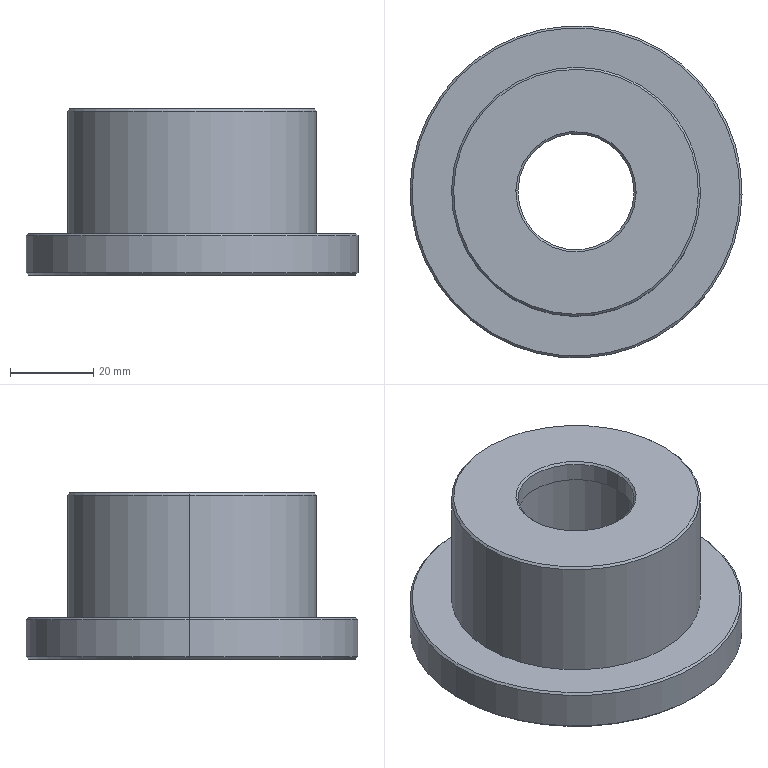Component | SolidWorks | HopperAssembly-1_20211103-210426-70669.STEP-1_-_-_-1.STEP-1_-_-_-4.STEP-1 | 1 solid | 34 faces | box 80 x 80 x 40 mm | volume 97628 mm3 | cylinder 16 | cone 10 | plane 8 | commonest cylinder face diameters 35 x6 39.6 x2 60 x2 80 x2 37 x2 28 x2
STEP:
#1=COLOUR_RGB('',0.7922,0.8196,0.9333);
#2=FILL_AREA_STYLE_COLOUR('',#1);
#3=FILL_AREA_STYLE('',(#2));
#4=SURFACE_STYLE_FILL_AREA(#3);
#5=SURFACE_SIDE_STYLE('',(#4));
#6=SURFACE_STYLE_USAGE(.BOTH.,#5);
#7=PRESENTATION_STYLE_ASSIGNMENT((#6));
#8=CARTESIAN_POINT('',(-116.904,33.244,9.945));
#9=VERTEX_POINT('',#8);
#10=CARTESIAN_POINT('',(-115.526,33.22,9.945));
#11=VERTEX_POINT('',#10);
#12=CARTESIAN_POINT('',(-116.215,33.232,9.945));
#13=DIRECTION('',(0.,0.,-1.));
#14=DIRECTION('',(-0.9998,0.01747,0.));
#15=AXIS2_PLACEMENT_3D('',#12,#13,#14);
#16=CIRCLE('',#15,0.689);
#17=EDGE_CURVE('',#9,#11,#16,.T.);
#18=ORIENTED_EDGE('',*,*,#17,.T.);
#19=CARTESIAN_POINT('',(-115.526,33.22,10.733));
#20=VERTEX_POINT('',#19);
#21=CARTESIAN_POINT('',(-115.526,33.22,10.93));
#22=DIRECTION('',(-0.,-0.,1.));
#23=VECTOR('',#22,39.37);
#24=LINE('',#21,#23);
#25=EDGE_CURVE('',#11,#20,#24,.T.);
#26=ORIENTED_EDGE('',*,*,#25,.T.);
#27=CARTESIAN_POINT('',(-116.904,33.244,10.733));
#28=VERTEX_POINT('',#27);
#29=CARTESIAN_POINT('',(-116.215,33.232,10.733));
#30=DIRECTION('',(-0.,-0.,1.));
#31=DIRECTION('',(-0.9998,0.01747,0.));
#32=AXIS2_PLACEMENT_3D('',#29,#30,#31);
#33=CIRCLE('',#32,0.689);
#34=EDGE_CURVE('',#20,#28,#33,.T.);
#35=ORIENTED_EDGE('',*,*,#34,.T.);
#36=CARTESIAN_POINT('',(-116.904,33.244,10.93));
#37=DIRECTION('',(-0.,-0.,1.));
#38=VECTOR('',#37,39.37);
#39=LINE('',#36,#38);
#40=EDGE_CURVE('',#9,#28,#39,.T.);
#41=ORIENTED_EDGE('',*,*,#40,.F.);
#42=EDGE_LOOP('',(#18,#26,#35,#41));
#43=FACE_OUTER_BOUND('',#42,.T.);
#44=CARTESIAN_POINT('',(-116.215,33.232,10.93));
#45=DIRECTION('',(-0.,-0.,1.));
#46=DIRECTION('',(-0.9998,0.01747,0.));
#47=AXIS2_PLACEMENT_3D('',#44,#45,#46);
#48=CYLINDRICAL_SURFACE('',#47,0.689);
#49=ADVANCED_FACE('',(#43),#48,.F.);
#50=CARTESIAN_POINT('',(-115.436,33.218,9.886));
#51=VERTEX_POINT('',#50);
#52=CARTESIAN_POINT('',(-116.995,33.245,9.886));
#53=VERTEX_POINT('',#52);
#54=CARTESIAN_POINT('',(-116.215,33.232,9.886));
#55=DIRECTION('',(-0.,-0.,1.));
#56=DIRECTION('',(-0.9998,0.01747,0.));
#57=AXIS2_PLACEMENT_3D('',#54,#55,#56);
#58=CIRCLE('',#57,0.7795);
#59=EDGE_CURVE('',#51,#53,#58,.T.);
#60=ORIENTED_EDGE('',*,*,#59,.F.);
#61=CARTESIAN_POINT('',(-115.436,33.218,9.945));
#62=VERTEX_POINT('',#61);
#63=CARTESIAN_POINT('',(-115.436,33.218,11.52));
#64=DIRECTION('',(-0.,-0.,1.));
#65=VECTOR('',#64,39.37);
#66=LINE('',#63,#65);
#67=EDGE_CURVE('',#51,#62,#66,.T.);
#68=ORIENTED_EDGE('',*,*,#67,.T.);
#69=CARTESIAN_POINT('',(-116.995,33.245,9.945));
#70=VERTEX_POINT('',#69);
#71=CARTESIAN_POINT('',(-116.215,33.232,9.945));
#72=DIRECTION('',(-0.,-0.,1.));
#73=DIRECTION('',(-0.9998,0.01747,0.));
#74=AXIS2_PLACEMENT_3D('',#71,#72,#73);
#75=CIRCLE('',#74,0.7795);
#76=EDGE_CURVE('',#62,#70,#75,.T.);
#77=ORIENTED_EDGE('',*,*,#76,.T.);
#78=CARTESIAN_POINT('',(-116.995,33.245,11.52));
#79=DIRECTION('',(-0.,-0.,1.));
#80=VECTOR('',#79,39.37);
#81=LINE('',#78,#80);
#82=EDGE_CURVE('',#53,#70,#81,.T.);
#83=ORIENTED_EDGE('',*,*,#82,.F.);
#84=EDGE_LOOP('',(#60,#68,#77,#83));
#85=FACE_OUTER_BOUND('',#84,.T.);
#86=CARTESIAN_POINT('',(-116.215,33.232,11.52));
#87=DIRECTION('',(-0.,-0.,1.));
#88=DIRECTION('',(-0.9998,0.01747,0.));
#89=AXIS2_PLACEMENT_3D('',#86,#87,#88);
#90=CYLINDRICAL_SURFACE('',#89,0.7795);
#91=ADVANCED_FACE('',(#85),#90,.F.);
#92=CARTESIAN_POINT('',(-117.77,33.259,9.749));
#93=VERTEX_POINT('',#92);
#94=CARTESIAN_POINT('',(-117.79,33.259,9.729));
#95=VERTEX_POINT('',#94);
#96=CARTESIAN_POINT('',(-117.77,33.259,9.749));
#97=DIRECTION('',(-0.707,0.01235,-0.7071));
#98=VECTOR('',#97,39.37);
#99=LINE('',#96,#98);
#100=EDGE_CURVE('',#93,#95,#99,.T.);
#101=ORIENTED_EDGE('',*,*,#100,.F.);
#102=CARTESIAN_POINT('',(-114.66,33.205,9.749));
#103=VERTEX_POINT('',#102);
#104=CARTESIAN_POINT('',(-116.215,33.232,9.749));
#105=DIRECTION('',(-0.,-0.,1.));
#106=DIRECTION('',(0.9998,-0.01747,0.));
#107=AXIS2_PLACEMENT_3D('',#104,#105,#106);
#108=CIRCLE('',#107,1.555);
#109=EDGE_CURVE('',#103,#93,#108,.T.);
#110=ORIENTED_EDGE('',*,*,#109,.F.);
#111=CARTESIAN_POINT('',(-114.641,33.204,9.729));
#112=VERTEX_POINT('',#111);
#113=CARTESIAN_POINT('',(-114.66,33.205,9.749));
#114=DIRECTION('',(0.707,-0.01235,-0.7071));
#115=VECTOR('',#114,39.37);
#116=LINE('',#113,#115);
#117=EDGE_CURVE('',#103,#112,#116,.T.);
#118=ORIENTED_EDGE('',*,*,#117,.T.);
#119=CARTESIAN_POINT('',(-116.215,33.232,9.729));
#120=DIRECTION('',(0.,0.,-1.));
#121=DIRECTION('',(0.9998,-0.01747,0.));
#122=AXIS2_PLACEMENT_3D('',#119,#120,#121);
#123=CIRCLE('',#122,1.575);
#124=EDGE_CURVE('',#95,#112,#123,.T.);
#125=ORIENTED_EDGE('',*,*,#124,.F.);
#126=EDGE_LOOP('',(#101,#110,#118,#125));
#127=FACE_OUTER_BOUND('',#126,.T.);
#128=CARTESIAN_POINT('',(-116.215,33.232,9.749));
#129=DIRECTION('',(0.,0.,-1.));
#130=DIRECTION('',(0.9998,-0.01747,0.));
#131=AXIS2_PLACEMENT_3D('',#128,#129,#130);
#132=CONICAL_SURFACE('',#131,1.555,0.7854);
#133=ADVANCED_FACE('',(#127),#132,.T.);
#134=CARTESIAN_POINT('',(-114.66,33.205,9.355));
#135=VERTEX_POINT('',#134);
#136=CARTESIAN_POINT('',(-114.641,33.204,9.375));
#137=VERTEX_POINT('',#136);
#138=CARTESIAN_POINT('',(-114.641,33.204,9.375));
#139=DIRECTION('',(0.707,-0.01235,0.7071));
#140=VECTOR('',#139,39.37);
#141=LINE('',#138,#140);
#142=EDGE_CURVE('',#135,#137,#141,.T.);
#143=ORIENTED_EDGE('',*,*,#142,.F.);
#144=CARTESIAN_POINT('',(-117.77,33.259,9.355));
#145=VERTEX_POINT('',#144);
#146=CARTESIAN_POINT('',(-116.215,33.232,9.355));
#147=DIRECTION('',(0.,0.,-1.));
#148=DIRECTION('',(-0.9998,0.01747,-0.));
#149=AXIS2_PLACEMENT_3D('',#146,#147,#148);
#150=CIRCLE('',#149,1.555);
#151=EDGE_CURVE('',#145,#135,#150,.T.);
#152=ORIENTED_EDGE('',*,*,#151,.F.);
#153=CARTESIAN_POINT('',(-117.79,33.259,9.375));
#154=VERTEX_POINT('',#153);
#155=CARTESIAN_POINT('',(-117.79,33.259,9.375));
#156=DIRECTION('',(-0.707,0.01235,0.7071));
#157=VECTOR('',#156,39.37);
#158=LINE('',#155,#157);
#159=EDGE_CURVE('',#145,#154,#158,.T.);
#160=ORIENTED_EDGE('',*,*,#159,.T.);
#161=CARTESIAN_POINT('',(-116.215,33.232,9.375));
#162=DIRECTION('',(-0.,-0.,1.));
#163=DIRECTION('',(-0.9998,0.01747,-0.));
#164=AXIS2_PLACEMENT_3D('',#161,#162,#163);
#165=CIRCLE('',#164,1.575);
#166=EDGE_CURVE('',#137,#154,#165,.T.);
#167=ORIENTED_EDGE('',*,*,#166,.F.);
#168=EDGE_LOOP('',(#143,#152,#160,#167));
#169=FACE_OUTER_BOUND('',#168,.T.);
#170=CARTESIAN_POINT('',(-116.215,33.232,9.375));
#171=DIRECTION('',(-0.,-0.,1.));
#172=DIRECTION('',(-0.9998,0.01747,-0.));
#173=AXIS2_PLACEMENT_3D('',#170,#171,#172);
#174=CONICAL_SURFACE('',#173,1.575,0.7854);
#175=ADVANCED_FACE('',(#169),#174,.T.);
#176=CARTESIAN_POINT('',(-115.664,33.222,10.91));
#177=VERTEX_POINT('',#176);
#178=CARTESIAN_POINT('',(-115.644,33.222,10.93));
#179=VERTEX_POINT('',#178);
#180=CARTESIAN_POINT('',(-115.664,33.222,10.91));
#181=DIRECTION('',(0.707,-0.01235,0.7071));
#182=VECTOR('',#181,39.37);
#183=LINE('',#180,#182);
#184=EDGE_CURVE('',#177,#179,#183,.T.);
#185=ORIENTED_EDGE('',*,*,#184,.F.);
#186=CARTESIAN_POINT('',(-116.766,33.241,10.91));
#187=VERTEX_POINT('',#186);
#188=CARTESIAN_POINT('',(-116.215,33.232,10.91));
#189=DIRECTION('',(-0.,-0.,1.));
#190=DIRECTION('',(0.9998,-0.01747,0.));
#191=AXIS2_PLACEMENT_3D('',#188,#189,#190);
#192=CIRCLE('',#191,0.5512);
#193=EDGE_CURVE('',#187,#177,#192,.T.);
#194=ORIENTED_EDGE('',*,*,#193,.F.);
#195=CARTESIAN_POINT('',(-116.786,33.242,10.93));
#196=VERTEX_POINT('',#195);
#197=CARTESIAN_POINT('',(-116.766,33.241,10.91));
#198=DIRECTION('',(-0.707,0.01235,0.7071));
#199=VECTOR('',#198,39.37);
#200=LINE('',#197,#199);
#201=EDGE_CURVE('',#187,#196,#200,.T.);
#202=ORIENTED_EDGE('',*,*,#201,.T.);
#203=CARTESIAN_POINT('',(-116.215,33.232,10.93));
#204=DIRECTION('',(0.,0.,-1.));
#205=DIRECTION('',(0.9998,-0.01747,0.));
#206=AXIS2_PLACEMENT_3D('',#203,#204,#205);
#207=CIRCLE('',#206,0.5709);
#208=EDGE_CURVE('',#179,#196,#207,.T.);
#209=ORIENTED_EDGE('',*,*,#208,.F.);
#210=EDGE_LOOP('',(#185,#194,#202,#209));
#211=FACE_OUTER_BOUND('',#210,.T.);
#212=CARTESIAN_POINT('',(-116.215,33.232,10.91));
#213=DIRECTION('',(-0.,-0.,1.));
#214=DIRECTION('',(-0.9998,0.01747,0.));
#215=AXIS2_PLACEMENT_3D('',#212,#213,#214);
#216=CONICAL_SURFACE('',#215,0.5512,0.7854);
#217=ADVANCED_FACE('',(#211),#216,.F.);
#218=CARTESIAN_POINT('',(-117.376,33.252,10.93));
#219=VERTEX_POINT('',#218);
#220=CARTESIAN_POINT('',(-117.396,33.252,10.91));
#221=VERTEX_POINT('',#220);
#222=CARTESIAN_POINT('',(-117.376,33.252,10.93));
#223=DIRECTION('',(-0.707,0.01235,-0.7071));
#224=VECTOR('',#223,39.37);
#225=LINE('',#222,#224);
#226=EDGE_CURVE('',#219,#221,#225,.T.);
#227=ORIENTED_EDGE('',*,*,#226,.F.);
#228=CARTESIAN_POINT('',(-115.054,33.211,10.93));
#229=VERTEX_POINT('',#228);
#230=CARTESIAN_POINT('',(-116.215,33.232,10.93));
#231=DIRECTION('',(-0.,-0.,1.));
#232=DIRECTION('',(0.9998,-0.01747,0.));
#233=AXIS2_PLACEMENT_3D('',#230,#231,#232);
#234=CIRCLE('',#233,1.161);
#235=EDGE_CURVE('',#229,#219,#234,.T.);
#236=ORIENTED_EDGE('',*,*,#235,.F.);
#237=CARTESIAN_POINT('',(-115.034,33.211,10.91));
#238=VERTEX_POINT('',#237);
#239=CARTESIAN_POINT('',(-115.054,33.211,10.93));
#240=DIRECTION('',(0.707,-0.01235,-0.7071));
#241=VECTOR('',#240,39.37);
#242=LINE('',#239,#241);
#243=EDGE_CURVE('',#229,#238,#242,.T.);
#244=ORIENTED_EDGE('',*,*,#243,.T.);
#245=CARTESIAN_POINT('',(-116.215,33.232,10.91));
#246=DIRECTION('',(0.,0.,-1.));
#247=DIRECTION('',(0.9998,-0.01747,0.));
#248=AXIS2_PLACEMENT_3D('',#245,#246,#247);
#249=CIRCLE('',#248,1.181);
#250=EDGE_CURVE('',#221,#238,#249,.T.);
#251=ORIENTED_EDGE('',*,*,#250,.F.);
#252=EDGE_LOOP('',(#227,#236,#244,#251));
#253=FACE_OUTER_BOUND('',#252,.T.);
#254=CARTESIAN_POINT('',(-116.215,33.232,10.93));
#255=DIRECTION('',(0.,0.,-1.));
#256=DIRECTION('',(0.9998,-0.01747,0.));
#257=AXIS2_PLACEMENT_3D('',#254,#255,#256);
#258=CONICAL_SURFACE('',#257,1.161,0.7854);
#259=ADVANCED_FACE('',(#253),#258,.T.);
#260=CARTESIAN_POINT('',(-116.904,33.244,9.375));
#261=VERTEX_POINT('',#260);
#262=CARTESIAN_POINT('',(-116.924,33.244,9.355));
#263=VERTEX_POINT('',#262);
#264=CARTESIAN_POINT('',(-116.924,33.244,9.355));
#265=DIRECTION('',(-0.707,0.01235,-0.7071));
#266=VECTOR('',#265,39.37);
#267=LINE('',#264,#266);
#268=EDGE_CURVE('',#261,#263,#267,.T.);
#269=ORIENTED_EDGE('',*,*,#268,.F.);
#270=CARTESIAN_POINT('',(-115.526,33.22,9.375));
#271=VERTEX_POINT('',#270);
#272=CARTESIAN_POINT('',(-116.215,33.232,9.375));
#273=DIRECTION('',(0.,0.,-1.));
#274=DIRECTION('',(-0.9998,0.01747,-0.));
#275=AXIS2_PLACEMENT_3D('',#272,#273,#274);
#276=CIRCLE('',#275,0.689);
#277=EDGE_CURVE('',#271,#261,#276,.T.);
#278=ORIENTED_EDGE('',*,*,#277,.F.);
#279=CARTESIAN_POINT('',(-115.507,33.219,9.355));
#280=VERTEX_POINT('',#279);
#281=CARTESIAN_POINT('',(-115.507,33.219,9.355));
#282=DIRECTION('',(0.707,-0.01235,-0.7071));
#283=VECTOR('',#282,39.37);
#284=LINE('',#281,#283);
#285=EDGE_CURVE('',#271,#280,#284,.T.);
#286=ORIENTED_EDGE('',*,*,#285,.T.);
#287=CARTESIAN_POINT('',(-116.215,33.232,9.355));
#288=DIRECTION('',(-0.,-0.,1.));
#289=DIRECTION('',(-0.9998,0.01747,-0.));
#290=AXIS2_PLACEMENT_3D('',#287,#288,#289);
#291=CIRCLE('',#290,0.7087);
#292=EDGE_CURVE('',#263,#280,#291,.T.);
#293=ORIENTED_EDGE('',*,*,#292,.F.);
#294=EDGE_LOOP('',(#269,#278,#286,#293));
#295=FACE_OUTER_BOUND('',#294,.T.);
#296=CARTESIAN_POINT('',(-116.215,33.232,9.355));
#297=DIRECTION('',(0.,0.,-1.));
#298=DIRECTION('',(0.9998,-0.01747,0.));
#299=AXIS2_PLACEMENT_3D('',#296,#297,#298);
#300=CONICAL_SURFACE('',#299,0.7087,0.7854);
#301=ADVANCED_FACE('',(#295),#300,.F.);
#302=CARTESIAN_POINT('',(-116.215,33.232,10.93));
#303=DIRECTION('',(0.,0.,-1.));
#304=DIRECTION('',(0.9998,-0.01747,0.));
#305=AXIS2_PLACEMENT_3D('',#302,#303,#304);
#306=CIRCLE('',#305,0.5709);
#307=EDGE_CURVE('',#196,#179,#306,.T.);
#308=ORIENTED_EDGE('',*,*,#307,.T.);
#309=ORIENTED_EDGE('',*,*,#208,.T.);
#310=EDGE_LOOP('',(#308,#309));
#311=FACE_BOUND('',#310,.T.);
#312=ORIENTED_EDGE('',*,*,#235,.T.);
#313=CARTESIAN_POINT('',(-116.215,33.232,10.93));
#314=DIRECTION('',(-0.,-0.,1.));
#315=DIRECTION('',(0.9998,-0.01747,0.));
#316=AXIS2_PLACEMENT_3D('',#313,#314,#315);
#317=CIRCLE('',#316,1.161);
#318=EDGE_CURVE('',#219,#229,#317,.T.);
#319=ORIENTED_EDGE('',*,*,#318,.T.);
#320=EDGE_LOOP('',(#312,#319));
#321=FACE_OUTER_BOUND('',#320,.T.);
#322=CARTESIAN_POINT('',(-116.225,32.681,10.93));
#323=DIRECTION('',(0.,0.,-1.));
#324=DIRECTION('',(-0.01747,-0.9998,-0.));
#325=AXIS2_PLACEMENT_3D('',#322,#323,#324);
#326=PLANE('',#325);
#327=ADVANCED_FACE('',(#311,#321),#326,.F.);
#328=CARTESIAN_POINT('',(-115.034,33.211,9.749));
#329=VERTEX_POINT('',#328);
#330=CARTESIAN_POINT('',(-115.034,33.211,10.93));
#331=DIRECTION('',(-0.,-0.,1.));
#332=VECTOR('',#331,39.37);
#333=LINE('',#330,#332);
#334=EDGE_CURVE('',#329,#238,#333,.T.);
#335=ORIENTED_EDGE('',*,*,#334,.F.);
#336=CARTESIAN_POINT('',(-117.396,33.252,9.749));
#337=VERTEX_POINT('',#336);
#338=CARTESIAN_POINT('',(-116.215,33.232,9.749));
#339=DIRECTION('',(-0.,-0.,1.));
#340=DIRECTION('',(-0.9998,0.01747,-0.));
#341=AXIS2_PLACEMENT_3D('',#338,#339,#340);
#342=CIRCLE('',#341,1.181);
#343=EDGE_CURVE('',#329,#337,#342,.T.);
#344=ORIENTED_EDGE('',*,*,#343,.T.);
#345=CARTESIAN_POINT('',(-117.396,33.252,10.93));
#346=DIRECTION('',(-0.,-0.,1.));
#347=VECTOR('',#346,39.37);
#348=LINE('',#345,#347);
#349=EDGE_CURVE('',#337,#221,#348,.T.);
#350=ORIENTED_EDGE('',*,*,#349,.T.);
#351=ORIENTED_EDGE('',*,*,#250,.T.);
#352=EDGE_LOOP('',(#335,#344,#350,#351));
#353=FACE_OUTER_BOUND('',#352,.T.);
#354=CARTESIAN_POINT('',(-116.215,33.232,10.93));
#355=DIRECTION('',(-0.,-0.,1.));
#356=DIRECTION('',(-0.9998,0.01747,-0.));
#357=AXIS2_PLACEMENT_3D('',#354,#355,#356);
#358=CYLINDRICAL_SURFACE('',#357,1.181);
#359=ADVANCED_FACE('',(#353),#358,.T.);
#360=CARTESIAN_POINT('',(-116.215,33.232,9.749));
#361=DIRECTION('',(-0.,-0.,1.));
#362=DIRECTION('',(-0.9998,0.01747,-0.));
#363=AXIS2_PLACEMENT_3D('',#360,#361,#362);
#364=CIRCLE('',#363,1.181);
#365=EDGE_CURVE('',#337,#329,#364,.T.);
#366=ORIENTED_EDGE('',*,*,#365,.F.);
#367=ORIENTED_EDGE('',*,*,#343,.F.);
#368=EDGE_LOOP('',(#366,#367));
#369=FACE_BOUND('',#368,.T.);
#370=ORIENTED_EDGE('',*,*,#109,.T.);
#371=CARTESIAN_POINT('',(-116.215,33.232,9.749));
#372=DIRECTION('',(-0.,-0.,1.));
#373=DIRECTION('',(0.9998,-0.01747,0.));
#374=AXIS2_PLACEMENT_3D('',#371,#372,#373);
#375=CIRCLE('',#374,1.555);
#376=EDGE_CURVE('',#93,#103,#375,.T.);
#377=ORIENTED_EDGE('',*,*,#376,.T.);
#378=EDGE_LOOP('',(#370,#377));
#379=FACE_OUTER_BOUND('',#378,.T.);
#380=CARTESIAN_POINT('',(-116.236,32.051,9.749));
#381=DIRECTION('',(0.,0.,-1.));
#382=DIRECTION('',(-0.01747,-0.9998,-0.));
#383=AXIS2_PLACEMENT_3D('',#380,#381,#382);
#384=PLANE('',#383);
#385=ADVANCED_FACE('',(#369,#379),#384,.F.);
#386=CARTESIAN_POINT('',(-114.641,33.204,10.93));
#387=DIRECTION('',(-0.,-0.,1.));
#388=VECTOR('',#387,39.37);
#389=LINE('',#386,#388);
#390=EDGE_CURVE('',#137,#112,#389,.T.);
#391=ORIENTED_EDGE('',*,*,#390,.F.);
#392=ORIENTED_EDGE('',*,*,#166,.T.);
#393=CARTESIAN_POINT('',(-117.79,33.259,10.93));
#394=DIRECTION('',(-0.,-0.,1.));
#395=VECTOR('',#394,39.37);
#396=LINE('',#393,#395);
#397=EDGE_CURVE('',#154,#95,#396,.T.);
#398=ORIENTED_EDGE('',*,*,#397,.T.);
#399=ORIENTED_EDGE('',*,*,#124,.T.);
#400=EDGE_LOOP('',(#391,#392,#398,#399));
#401=FACE_OUTER_BOUND('',#400,.T.);
#402=CARTESIAN_POINT('',(-116.215,33.232,10.93));
#403=DIRECTION('',(-0.,-0.,1.));
#404=DIRECTION('',(-0.9998,0.01747,-0.));
#405=AXIS2_PLACEMENT_3D('',#402,#403,#404);
#406=CYLINDRICAL_SURFACE('',#405,1.575);
#407=ADVANCED_FACE('',(#401),#406,.T.);
#408=CARTESIAN_POINT('',(-116.215,33.232,9.355));
#409=DIRECTION('',(-0.,-0.,1.));
#410=DIRECTION('',(-0.9998,0.01747,-0.));
#411=AXIS2_PLACEMENT_3D('',#408,#409,#410);
#412=CIRCLE('',#411,0.7087);
#413=EDGE_CURVE('',#280,#263,#412,.T.);
#414=ORIENTED_EDGE('',*,*,#413,.T.);
#415=ORIENTED_EDGE('',*,*,#292,.T.);
#416=EDGE_LOOP('',(#414,#415));
#417=FACE_BOUND('',#416,.T.);
#418=ORIENTED_EDGE('',*,*,#151,.T.);
#419=CARTESIAN_POINT('',(-116.215,33.232,9.355));
#420=DIRECTION('',(0.,0.,-1.));
#421=DIRECTION('',(-0.9998,0.01747,-0.));
#422=AXIS2_PLACEMENT_3D('',#419,#420,#421);
#423=CIRCLE('',#422,1.555);
#424=EDGE_CURVE('',#135,#145,#423,.T.);
#425=ORIENTED_EDGE('',*,*,#424,.T.);
#426=EDGE_LOOP('',(#418,#425));
#427=FACE_OUTER_BOUND('',#426,.T.);
#428=CARTESIAN_POINT('',(-116.227,32.543,9.355));
#429=DIRECTION('',(-0.,-0.,1.));
#430=DIRECTION('',(-0.9998,0.01747,-0.));
#431=AXIS2_PLACEMENT_3D('',#428,#429,#430);
#432=PLANE('',#431);
#433=ADVANCED_FACE('',(#417,#427),#432,.F.);
#434=CARTESIAN_POINT('',(-115.526,33.22,9.485));
#435=VERTEX_POINT('',#434);
#436=CARTESIAN_POINT('',(-115.526,33.22,10.93));
#437=DIRECTION('',(-0.,-0.,1.));
#438=VECTOR('',#437,39.37);
#439=LINE('',#436,#438);
#440=EDGE_CURVE('',#271,#435,#439,.T.);
#441=ORIENTED_EDGE('',*,*,#440,.F.);
#442=ORIENTED_EDGE('',*,*,#277,.T.);
#443=CARTESIAN_POINT('',(-116.904,33.244,9.485));
#444=VERTEX_POINT('',#443);
#445=CARTESIAN_POINT('',(-116.904,33.244,10.93));
#446=DIRECTION('',(-0.,-0.,1.));
#447=VECTOR('',#446,39.37);
#448=LINE('',#445,#447);
#449=EDGE_CURVE('',#261,#444,#448,.T.);
#450=ORIENTED_EDGE('',*,*,#449,.T.);
#451=CARTESIAN_POINT('',(-116.215,33.232,9.485));
#452=DIRECTION('',(-0.,-0.,1.));
#453=DIRECTION('',(-0.9998,0.01747,-0.));
#454=AXIS2_PLACEMENT_3D('',#451,#452,#453);
#455=CIRCLE('',#454,0.689);
#456=EDGE_CURVE('',#444,#435,#455,.T.);
#457=ORIENTED_EDGE('',*,*,#456,.T.);
#458=EDGE_LOOP('',(#441,#442,#450,#457));
#459=FACE_OUTER_BOUND('',#458,.T.);
#460=CARTESIAN_POINT('',(-116.215,33.232,10.93));
#461=DIRECTION('',(-0.,-0.,1.));
#462=DIRECTION('',(-0.9998,0.01747,0.));
#463=AXIS2_PLACEMENT_3D('',#460,#461,#462);
#464=CYLINDRICAL_SURFACE('',#463,0.689);
#465=ADVANCED_FACE('',(#459),#464,.F.);
#466=ORIENTED_EDGE('',*,*,#456,.F.);
#467=CARTESIAN_POINT('',(-116.215,33.232,9.485));
#468=DIRECTION('',(-0.,-0.,1.));
#469=DIRECTION('',(-0.9998,0.01747,-0.));
#470=AXIS2_PLACEMENT_3D('',#467,#468,#469);
#471=CIRCLE('',#470,0.689);
#472=EDGE_CURVE('',#435,#444,#471,.T.);
#473=ORIENTED_EDGE('',*,*,#472,.F.);
#474=EDGE_LOOP('',(#466,#473));
#475=FACE_BOUND('',#474,.T.);
#476=CARTESIAN_POINT('',(-116.943,33.245,9.485));
#477=VERTEX_POINT('',#476);
#478=CARTESIAN_POINT('',(-115.487,33.219,9.485));
#479=VERTEX_POINT('',#478);
#480=CARTESIAN_POINT('',(-116.215,33.232,9.485));
#481=DIRECTION('',(-0.,-0.,1.));
#482=DIRECTION('',(-0.9998,0.01747,-0.));
#483=AXIS2_PLACEMENT_3D('',#480,#481,#482);
#484=CIRCLE('',#483,0.7283);
#485=EDGE_CURVE('',#477,#479,#484,.T.);
#486=ORIENTED_EDGE('',*,*,#485,.T.);
#487=CARTESIAN_POINT('',(-116.215,33.232,9.485));
#488=DIRECTION('',(-0.,-0.,1.));
#489=DIRECTION('',(-0.9998,0.01747,-0.));
#490=AXIS2_PLACEMENT_3D('',#487,#488,#489);
#491=CIRCLE('',#490,0.7283);
#492=EDGE_CURVE('',#479,#477,#491,.T.);
#493=ORIENTED_EDGE('',*,*,#492,.T.);
#494=EDGE_LOOP('',(#486,#493));
#495=FACE_OUTER_BOUND('',#494,.T.);
#496=CARTESIAN_POINT('',(-116.228,32.504,9.485));
#497=DIRECTION('',(0.,0.,-1.));
#498=DIRECTION('',(-0.01747,-0.9998,-0.));
#499=AXIS2_PLACEMENT_3D('',#496,#497,#498);
#500=PLANE('',#499);
#501=ADVANCED_FACE('',(#475,#495),#500,.F.);
#502=CARTESIAN_POINT('',(-115.487,33.219,9.552));
#503=VERTEX_POINT('',#502);
#504=CARTESIAN_POINT('',(-115.487,33.219,10.93));
#505=DIRECTION('',(-0.,-0.,1.));
#506=VECTOR('',#505,39.37);
#507=LINE('',#504,#506);
#508=EDGE_CURVE('',#479,#503,#507,.T.);
#509=ORIENTED_EDGE('',*,*,#508,.F.);
#510=ORIENTED_EDGE('',*,*,#485,.F.);
#511=CARTESIAN_POINT('',(-116.943,33.245,9.552));
#512=VERTEX_POINT('',#511);
#513=CARTESIAN_POINT('',(-116.943,33.245,10.93));
#514=DIRECTION('',(-0.,-0.,1.));
#515=VECTOR('',#514,39.37);
#516=LINE('',#513,#515);
#517=EDGE_CURVE('',#477,#512,#516,.T.);
#518=ORIENTED_EDGE('',*,*,#517,.T.);
#519=CARTESIAN_POINT('',(-116.215,33.232,9.552));
#520=DIRECTION('',(-0.,-0.,1.));
#521=DIRECTION('',(-0.9998,0.01747,-0.));
#522=AXIS2_PLACEMENT_3D('',#519,#520,#521);
#523=CIRCLE('',#522,0.7283);
#524=EDGE_CURVE('',#512,#503,#523,.T.);
#525=ORIENTED_EDGE('',*,*,#524,.T.);
#526=EDGE_LOOP('',(#509,#510,#518,#525));
#527=FACE_OUTER_BOUND('',#526,.T.);
#528=CARTESIAN_POINT('',(-116.215,33.232,10.93));
#529=DIRECTION('',(-0.,-0.,1.));
#530=DIRECTION('',(-0.9998,0.01747,0.));
#531=AXIS2_PLACEMENT_3D('',#528,#529,#530);
#532=CYLINDRICAL_SURFACE('',#531,0.7283);
#533=ADVANCED_FACE('',(#527),#532,.F.);
#534=CARTESIAN_POINT('',(-116.904,33.244,9.552));
#535=VERTEX_POINT('',#534);
#536=CARTESIAN_POINT('',(-115.526,33.22,9.552));
#537=VERTEX_POINT('',#536);
#538=CARTESIAN_POINT('',(-116.215,33.232,9.552));
#539=DIRECTION('',(-0.,-0.,1.));
#540=DIRECTION('',(-0.9998,0.01747,-0.));
#541=AXIS2_PLACEMENT_3D('',#538,#539,#540);
#542=CIRCLE('',#541,0.689);
#543=EDGE_CURVE('',#535,#537,#542,.T.);
#544=ORIENTED_EDGE('',*,*,#543,.T.);
#545=CARTESIAN_POINT('',(-116.215,33.232,9.552));
#546=DIRECTION('',(-0.,-0.,1.));
#547=DIRECTION('',(-0.9998,0.01747,-0.));
#548=AXIS2_PLACEMENT_3D('',#545,#546,#547);
#549=CIRCLE('',#548,0.689);
#550=EDGE_CURVE('',#537,#535,#549,.T.);
#551=ORIENTED_EDGE('',*,*,#550,.T.);
#552=EDGE_LOOP('',(#544,#551));
#553=FACE_BOUND('',#552,.T.);
#554=ORIENTED_EDGE('',*,*,#524,.F.);
#555=CARTESIAN_POINT('',(-116.215,33.232,9.552));
#556=DIRECTION('',(-0.,-0.,1.));
#557=DIRECTION('',(-0.9998,0.01747,-0.));
#558=AXIS2_PLACEMENT_3D('',#555,#556,#557);
#559=CIRCLE('',#558,0.7283);
#560=EDGE_CURVE('',#503,#512,#559,.T.);
#561=ORIENTED_EDGE('',*,*,#560,.F.);
#562=EDGE_LOOP('',(#554,#561));
#563=FACE_OUTER_BOUND('',#562,.T.);
#564=CARTESIAN_POINT('',(-116.227,32.543,9.552));
#565=DIRECTION('',(-0.,-0.,1.));
#566=DIRECTION('',(-0.9998,0.01747,-0.));
#567=AXIS2_PLACEMENT_3D('',#564,#565,#566);
#568=PLANE('',#567);
#569=ADVANCED_FACE('',(#553,#563),#568,.F.);
#570=CARTESIAN_POINT('',(-116.904,33.244,9.886));
#571=VERTEX_POINT('',#570);
#572=CARTESIAN_POINT('',(-116.904,33.244,10.93));
#573=DIRECTION('',(-0.,-0.,1.));
#574=VECTOR('',#573,39.37);
#575=LINE('',#572,#574);
#576=EDGE_CURVE('',#535,#571,#575,.T.);
#577=ORIENTED_EDGE('',*,*,#576,.T.);
#578=CARTESIAN_POINT('',(-115.526,33.22,9.886));
#579=VERTEX_POINT('',#578);
#580=CARTESIAN_POINT('',(-116.215,33.232,9.886));
#581=DIRECTION('',(-0.,-0.,1.));
#582=DIRECTION('',(0.9998,-0.01747,0.));
#583=AXIS2_PLACEMENT_3D('',#580,#581,#582);
#584=CIRCLE('',#583,0.689);
#585=EDGE_CURVE('',#571,#579,#584,.T.);
#586=ORIENTED_EDGE('',*,*,#585,.T.);
#587=CARTESIAN_POINT('',(-115.526,33.22,10.93));
#588=DIRECTION('',(-0.,-0.,1.));
#589=VECTOR('',#588,39.37);
#590=LINE('',#587,#589);
#591=EDGE_CURVE('',#537,#579,#590,.T.);
#592=ORIENTED_EDGE('',*,*,#591,.F.);
#593=ORIENTED_EDGE('',*,*,#543,.F.);
#594=EDGE_LOOP('',(#577,#586,#592,#593));
#595=FACE_OUTER_BOUND('',#594,.T.);
#596=CARTESIAN_POINT('',(-116.215,33.232,10.93));
#597=DIRECTION('',(-0.,-0.,1.));
#598=DIRECTION('',(-0.9998,0.01747,0.));
#599=AXIS2_PLACEMENT_3D('',#596,#597,#598);
#600=CYLINDRICAL_SURFACE('',#599,0.689);
#601=ADVANCED_FACE('',(#595),#600,.F.);
#602=CARTESIAN_POINT('',(-115.664,33.222,10.733));
#603=VERTEX_POINT('',#602);
#604=CARTESIAN_POINT('',(-115.664,33.222,10.93));
#605=DIRECTION('',(-0.,-0.,1.));
#606=VECTOR('',#605,39.37);
#607=LINE('',#604,#606);
#608=EDGE_CURVE('',#603,#177,#607,.T.);
#609=ORIENTED_EDGE('',*,*,#608,.F.);
#610=CARTESIAN_POINT('',(-116.766,33.241,10.733));
#611=VERTEX_POINT('',#610);
#612=CARTESIAN_POINT('',(-116.215,33.232,10.733));
#613=DIRECTION('',(0.,0.,-1.));
#614=DIRECTION('',(-0.9998,0.01747,0.));
#615=AXIS2_PLACEMENT_3D('',#612,#613,#614);
#616=CIRCLE('',#615,0.5512);
#617=EDGE_CURVE('',#603,#611,#616,.T.);
#618=ORIENTED_EDGE('',*,*,#617,.T.);
#619=CARTESIAN_POINT('',(-116.766,33.241,10.93));
#620=DIRECTION('',(-0.,-0.,1.));
#621=VECTOR('',#620,39.37);
#622=LINE('',#619,#621);
#623=EDGE_CURVE('',#611,#187,#622,.T.);
#624=ORIENTED_EDGE('',*,*,#623,.T.);
#625=ORIENTED_EDGE('',*,*,#193,.T.);
#626=EDGE_LOOP('',(#609,#618,#624,#625));
#627=FACE_OUTER_BOUND('',#626,.T.);
#628=CARTESIAN_POINT('',(-116.215,33.232,10.93));
#629=DIRECTION('',(-0.,-0.,1.));
#630=DIRECTION('',(-0.9998,0.01747,0.));
#631=AXIS2_PLACEMENT_3D('',#628,#629,#630);
#632=CYLINDRICAL_SURFACE('',#631,0.5512);
#633=ADVANCED_FACE('',(#627),#632,.F.);
#634=ORIENTED_EDGE('',*,*,#623,.F.);
#635=CARTESIAN_POINT('',(-116.215,33.232,10.733));
#636=DIRECTION('',(0.,0.,-1.));
#637=DIRECTION('',(-0.9998,0.01747,0.));
#638=AXIS2_PLACEMENT_3D('',#635,#636,#637);
#639=CIRCLE('',#638,0.5512);
#640=EDGE_CURVE('',#611,#603,#639,.T.);
#641=ORIENTED_EDGE('',*,*,#640,.T.);
#642=ORIENTED_EDGE('',*,*,#608,.T.);
#643=CARTESIAN_POINT('',(-116.215,33.232,10.91));
#644=DIRECTION('',(-0.,-0.,1.));
#645=DIRECTION('',(0.9998,-0.01747,0.));
#646=AXIS2_PLACEMENT_3D('',#643,#644,#645);
#647=CIRCLE('',#646,0.5512);
#648=EDGE_CURVE('',#177,#187,#647,.T.);
#649=ORIENTED_EDGE('',*,*,#648,.T.);
#650=EDGE_LOOP('',(#634,#641,#642,#649));
#651=FACE_OUTER_BOUND('',#650,.T.);
#652=CARTESIAN_POINT('',(-116.215,33.232,10.93));
#653=DIRECTION('',(-0.,-0.,1.));
#654=DIRECTION('',(-0.9998,0.01747,0.));
#655=AXIS2_PLACEMENT_3D('',#652,#653,#654);
#656=CYLINDRICAL_SURFACE('',#655,0.5512);
#657=ADVANCED_FACE('',(#651),#656,.F.);
#658=ORIENTED_EDGE('',*,*,#591,.T.);
#659=CARTESIAN_POINT('',(-116.215,33.232,9.886));
#660=DIRECTION('',(-0.,-0.,1.));
#661=DIRECTION('',(0.9998,-0.01747,0.));
#662=AXIS2_PLACEMENT_3D('',#659,#660,#661);
#663=CIRCLE('',#662,0.689);
#664=EDGE_CURVE('',#579,#571,#663,.T.);
#665=ORIENTED_EDGE('',*,*,#664,.T.);
#666=ORIENTED_EDGE('',*,*,#576,.F.);
#667=ORIENTED_EDGE('',*,*,#550,.F.);
#668=EDGE_LOOP('',(#658,#665,#666,#667));
#669=FACE_OUTER_BOUND('',#668,.T.);
#670=CARTESIAN_POINT('',(-116.215,33.232,10.93));
#671=DIRECTION('',(-0.,-0.,1.));
#672=DIRECTION('',(-0.9998,0.01747,0.));
#673=AXIS2_PLACEMENT_3D('',#670,#671,#672);
#674=CYLINDRICAL_SURFACE('',#673,0.689);
#675=ADVANCED_FACE('',(#669),#674,.F.);
#676=ORIENTED_EDGE('',*,*,#492,.F.);
#677=ORIENTED_EDGE('',*,*,#508,.T.);
#678=ORIENTED_EDGE('',*,*,#560,.T.);
#679=ORIENTED_EDGE('',*,*,#517,.F.);
#680=EDGE_LOOP('',(#676,#677,#678,#679));
#681=FACE_OUTER_BOUND('',#680,.T.);
#682=CARTESIAN_POINT('',(-116.215,33.232,10.93));
#683=DIRECTION('',(-0.,-0.,1.));
#684=DIRECTION('',(-0.9998,0.01747,0.));
#685=AXIS2_PLACEMENT_3D('',#682,#683,#684);
#686=CYLINDRICAL_SURFACE('',#685,0.7283);
#687=ADVANCED_FACE('',(#681),#686,.F.);
#688=CARTESIAN_POINT('',(-116.215,33.232,9.375));
#689=DIRECTION('',(0.,0.,-1.));
#690=DIRECTION('',(-0.9998,0.01747,-0.));
#691=AXIS2_PLACEMENT_3D('',#688,#689,#690);
#692=CIRCLE('',#691,0.689);
#693=EDGE_CURVE('',#261,#271,#692,.T.);
#694=ORIENTED_EDGE('',*,*,#693,.T.);
#695=ORIENTED_EDGE('',*,*,#440,.T.);
#696=ORIENTED_EDGE('',*,*,#472,.T.);
#697=ORIENTED_EDGE('',*,*,#449,.F.);
#698=EDGE_LOOP('',(#694,#695,#696,#697));
#699=FACE_OUTER_BOUND('',#698,.T.);
#700=CARTESIAN_POINT('',(-116.215,33.232,10.93));
#701=DIRECTION('',(-0.,-0.,1.));
#702=DIRECTION('',(-0.9998,0.01747,0.));
#703=AXIS2_PLACEMENT_3D('',#700,#701,#702);
#704=CYLINDRICAL_SURFACE('',#703,0.689);
#705=ADVANCED_FACE('',(#699),#704,.F.);
#706=CARTESIAN_POINT('',(-116.215,33.232,9.375));
#707=DIRECTION('',(-0.,-0.,1.));
#708=DIRECTION('',(-0.9998,0.01747,-0.));
#709=AXIS2_PLACEMENT_3D('',#706,#707,#708);
#710=CIRCLE('',#709,1.575);
#711=EDGE_CURVE('',#154,#137,#710,.T.);
#712=ORIENTED_EDGE('',*,*,#711,.T.);
#713=ORIENTED_EDGE('',*,*,#390,.T.);
#714=CARTESIAN_POINT('',(-116.215,33.232,9.729));
#715=DIRECTION('',(0.,0.,-1.));
#716=DIRECTION('',(0.9998,-0.01747,0.));
#717=AXIS2_PLACEMENT_3D('',#714,#715,#716);
#718=CIRCLE('',#717,1.575);
#719=EDGE_CURVE('',#112,#95,#718,.T.);
#720=ORIENTED_EDGE('',*,*,#719,.T.);
#721=ORIENTED_EDGE('',*,*,#397,.F.);
#722=EDGE_LOOP('',(#712,#713,#720,#721));
#723=FACE_OUTER_BOUND('',#722,.T.);
#724=CARTESIAN_POINT('',(-116.215,33.232,10.93));
#725=DIRECTION('',(-0.,-0.,1.));
#726=DIRECTION('',(-0.9998,0.01747,-0.));
#727=AXIS2_PLACEMENT_3D('',#724,#725,#726);
#728=CYLINDRICAL_SURFACE('',#727,1.575);
#729=ADVANCED_FACE('',(#723),#728,.T.);
#730=ORIENTED_EDGE('',*,*,#365,.T.);
#731=ORIENTED_EDGE('',*,*,#334,.T.);
#732=CARTESIAN_POINT('',(-116.215,33.232,10.91));
#733=DIRECTION('',(0.,0.,-1.));
#734=DIRECTION('',(0.9998,-0.01747,0.));
#735=AXIS2_PLACEMENT_3D('',#732,#733,#734);
#736=CIRCLE('',#735,1.181);
#737=EDGE_CURVE('',#238,#221,#736,.T.);
#738=ORIENTED_EDGE('',*,*,#737,.T.);
#739=ORIENTED_EDGE('',*,*,#349,.F.);
#740=EDGE_LOOP('',(#730,#731,#738,#739));
#741=FACE_OUTER_BOUND('',#740,.T.);
#742=CARTESIAN_POINT('',(-116.215,33.232,10.93));
#743=DIRECTION('',(-0.,-0.,1.));
#744=DIRECTION('',(-0.9998,0.01747,-0.));
#745=AXIS2_PLACEMENT_3D('',#742,#743,#744);
#746=CYLINDRICAL_SURFACE('',#745,1.181);
#747=ADVANCED_FACE('',(#741),#746,.T.);
#748=ORIENTED_EDGE('',*,*,#693,.F.);
#749=ORIENTED_EDGE('',*,*,#268,.T.);
#750=ORIENTED_EDGE('',*,*,#413,.F.);
#751=ORIENTED_EDGE('',*,*,#285,.F.);
#752=EDGE_LOOP('',(#748,#749,#750,#751));
#753=FACE_OUTER_BOUND('',#752,.T.);
#754=CARTESIAN_POINT('',(-116.215,33.232,9.355));
#755=DIRECTION('',(0.,0.,-1.));
#756=DIRECTION('',(0.9998,-0.01747,0.));
#757=AXIS2_PLACEMENT_3D('',#754,#755,#756);
#758=CONICAL_SURFACE('',#757,0.7087,0.7854);
#759=ADVANCED_FACE('',(#753),#758,.F.);
#760=ORIENTED_EDGE('',*,*,#318,.F.);
#761=ORIENTED_EDGE('',*,*,#226,.T.);
#762=ORIENTED_EDGE('',*,*,#737,.F.);
#763=ORIENTED_EDGE('',*,*,#243,.F.);
#764=EDGE_LOOP('',(#760,#761,#762,#763));
#765=FACE_OUTER_BOUND('',#764,.T.);
#766=CARTESIAN_POINT('',(-116.215,33.232,10.93));
#767=DIRECTION('',(0.,0.,-1.));
#768=DIRECTION('',(0.9998,-0.01747,0.));
#769=AXIS2_PLACEMENT_3D('',#766,#767,#768);
#770=CONICAL_SURFACE('',#769,1.161,0.7854);
#771=ADVANCED_FACE('',(#765),#770,.T.);
#772=ORIENTED_EDGE('',*,*,#648,.F.);
#773=ORIENTED_EDGE('',*,*,#184,.T.);
#774=ORIENTED_EDGE('',*,*,#307,.F.);
#775=ORIENTED_EDGE('',*,*,#201,.F.);
#776=EDGE_LOOP('',(#772,#773,#774,#775));
#777=FACE_OUTER_BOUND('',#776,.T.);
#778=CARTESIAN_POINT('',(-116.215,33.232,10.91));
#779=DIRECTION('',(-0.,-0.,1.));
#780=DIRECTION('',(-0.9998,0.01747,0.));
#781=AXIS2_PLACEMENT_3D('',#778,#779,#780);
#782=CONICAL_SURFACE('',#781,0.5512,0.7854);
#783=ADVANCED_FACE('',(#777),#782,.F.);
#784=ORIENTED_EDGE('',*,*,#424,.F.);
#785=ORIENTED_EDGE('',*,*,#142,.T.);
#786=ORIENTED_EDGE('',*,*,#711,.F.);
#787=ORIENTED_EDGE('',*,*,#159,.F.);
#788=EDGE_LOOP('',(#784,#785,#786,#787));
#789=FACE_OUTER_BOUND('',#788,.T.);
#790=CARTESIAN_POINT('',(-116.215,33.232,9.375));
#791=DIRECTION('',(-0.,-0.,1.));
#792=DIRECTION('',(-0.9998,0.01747,-0.));
#793=AXIS2_PLACEMENT_3D('',#790,#791,#792);
#794=CONICAL_SURFACE('',#793,1.575,0.7854);
#795=ADVANCED_FACE('',(#789),#794,.T.);
#796=ORIENTED_EDGE('',*,*,#376,.F.);
#797=ORIENTED_EDGE('',*,*,#100,.T.);
#798=ORIENTED_EDGE('',*,*,#719,.F.);
#799=ORIENTED_EDGE('',*,*,#117,.F.);
#800=EDGE_LOOP('',(#796,#797,#798,#799));
#801=FACE_OUTER_BOUND('',#800,.T.);
#802=CARTESIAN_POINT('',(-116.215,33.232,9.749));
#803=DIRECTION('',(0.,0.,-1.));
#804=DIRECTION('',(0.9998,-0.01747,0.));
#805=AXIS2_PLACEMENT_3D('',#802,#803,#804);
#806=CONICAL_SURFACE('',#805,1.555,0.7854);
#807=ADVANCED_FACE('',(#801),#806,.T.);
#808=CARTESIAN_POINT('',(-116.215,33.232,9.945));
#809=DIRECTION('',(-0.,-0.,1.));
#810=DIRECTION('',(-0.9998,0.01747,0.));
#811=AXIS2_PLACEMENT_3D('',#808,#809,#810);
#812=CIRCLE('',#811,0.7795);
#813=EDGE_CURVE('',#70,#62,#812,.T.);
#814=ORIENTED_EDGE('',*,*,#813,.F.);
#815=ORIENTED_EDGE('',*,*,#76,.F.);
#816=EDGE_LOOP('',(#814,#815));
#817=FACE_OUTER_BOUND('',#816,.T.);
#818=ORIENTED_EDGE('',*,*,#17,.F.);
#819=CARTESIAN_POINT('',(-116.215,33.232,9.945));
#820=DIRECTION('',(0.,0.,-1.));
#821=DIRECTION('',(-0.9998,0.01747,0.));
#822=AXIS2_PLACEMENT_3D('',#819,#820,#821);
#823=CIRCLE('',#822,0.689);
#824=EDGE_CURVE('',#11,#9,#823,.T.);
#825=ORIENTED_EDGE('',*,*,#824,.F.);
#826=EDGE_LOOP('',(#818,#825));
#827=FACE_BOUND('',#826,.T.);
#828=CARTESIAN_POINT('',(-116.995,33.245,9.945));
#829=DIRECTION('',(-0.,-0.,1.));
#830=DIRECTION('',(-0.9998,0.01747,-0.));
#831=AXIS2_PLACEMENT_3D('',#828,#829,#830);
#832=PLANE('',#831);
#833=ADVANCED_FACE('',(#817,#827),#832,.F.);
#834=CARTESIAN_POINT('',(-116.215,33.232,9.886));
#835=DIRECTION('',(-0.,-0.,1.));
#836=DIRECTION('',(-0.9998,0.01747,0.));
#837=AXIS2_PLACEMENT_3D('',#834,#835,#836);
#838=CIRCLE('',#837,0.7795);
#839=EDGE_CURVE('',#53,#51,#838,.T.);
#840=ORIENTED_EDGE('',*,*,#839,.T.);
#841=ORIENTED_EDGE('',*,*,#59,.T.);
#842=EDGE_LOOP('',(#840,#841));
#843=FACE_OUTER_BOUND('',#842,.T.);
#844=ORIENTED_EDGE('',*,*,#664,.F.);
#845=ORIENTED_EDGE('',*,*,#585,.F.);
#846=EDGE_LOOP('',(#844,#845));
#847=FACE_BOUND('',#846,.T.);
#848=CARTESIAN_POINT('',(-116.9,33.244,9.886));
#849=DIRECTION('',(0.,0.,-1.));
#850=DIRECTION('',(0.9998,-0.01747,0.));
#851=AXIS2_PLACEMENT_3D('',#848,#849,#850);
#852=PLANE('',#851);
#853=ADVANCED_FACE('',(#843,#847),#852,.F.);
#854=ORIENTED_EDGE('',*,*,#67,.F.);
#855=ORIENTED_EDGE('',*,*,#839,.F.);
#856=ORIENTED_EDGE('',*,*,#82,.T.);
#857=ORIENTED_EDGE('',*,*,#813,.T.);
#858=EDGE_LOOP('',(#854,#855,#856,#857));
#859=FACE_OUTER_BOUND('',#858,.T.);
#860=CARTESIAN_POINT('',(-116.215,33.232,11.52));
#861=DIRECTION('',(-0.,-0.,1.));
#862=DIRECTION('',(-0.9998,0.01747,0.));
#863=AXIS2_PLACEMENT_3D('',#860,#861,#862);
#864=CYLINDRICAL_SURFACE('',#863,0.7795);
#865=ADVANCED_FACE('',(#859),#864,.F.);
#866=ORIENTED_EDGE('',*,*,#25,.F.);
#867=ORIENTED_EDGE('',*,*,#824,.T.);
#868=ORIENTED_EDGE('',*,*,#40,.T.);
#869=CARTESIAN_POINT('',(-116.215,33.232,10.733));
#870=DIRECTION('',(-0.,-0.,1.));
#871=DIRECTION('',(-0.9998,0.01747,0.));
#872=AXIS2_PLACEMENT_3D('',#869,#870,#871);
#873=CIRCLE('',#872,0.689);
#874=EDGE_CURVE('',#28,#20,#873,.T.);
#875=ORIENTED_EDGE('',*,*,#874,.T.);
#876=EDGE_LOOP('',(#866,#867,#868,#875));
#877=FACE_OUTER_BOUND('',#876,.T.);
#878=CARTESIAN_POINT('',(-116.215,33.232,10.93));
#879=DIRECTION('',(-0.,-0.,1.));
#880=DIRECTION('',(-0.9998,0.01747,0.));
#881=AXIS2_PLACEMENT_3D('',#878,#879,#880);
#882=CYLINDRICAL_SURFACE('',#881,0.689);
#883=ADVANCED_FACE('',(#877),#882,.F.);
#884=ORIENTED_EDGE('',*,*,#874,.F.);
#885=ORIENTED_EDGE('',*,*,#34,.F.);
#886=EDGE_LOOP('',(#884,#885));
#887=FACE_OUTER_BOUND('',#886,.T.);
#888=ORIENTED_EDGE('',*,*,#640,.F.);
#889=ORIENTED_EDGE('',*,*,#617,.F.);
#890=EDGE_LOOP('',(#888,#889));
#891=FACE_BOUND('',#890,.T.);
#892=CARTESIAN_POINT('',(-116.904,33.244,10.733));
#893=DIRECTION('',(-0.,-0.,1.));
#894=DIRECTION('',(-0.9998,0.01747,-0.));
#895=AXIS2_PLACEMENT_3D('',#892,#893,#894);
#896=PLANE('',#895);
#897=ADVANCED_FACE('',(#887,#891),#896,.F.);
#898=CLOSED_SHELL('',(#49,#91,#133,#175,#217,#259,#301,#327,#359,#385,#407,#433,#465,#501,#533,#569,#601,#633,#657,#675,#687,#705,#729,#747,#759,#771,#783,#795,#807,#833,#853,#865,#883,#897));
#899=MANIFOLD_SOLID_BREP('',#898);
#900=STYLED_ITEM('',(#7),#899);
#901=(LENGTH_UNIT()NAMED_UNIT(*)SI_UNIT($,.METRE.));
#902=LENGTH_MEASURE_WITH_UNIT(LENGTH_MEASURE(0.0254),#901);
#903=DIMENSIONAL_EXPONENTS(1.,0.,0.,0.,0.,0.,0.);
#904=(CONVERSION_BASED_UNIT('',#902)LENGTH_UNIT()NAMED_UNIT(#903));
#905=UNCERTAINTY_MEASURE_WITH_UNIT(LENGTH_MEASURE(0.00001),#904,'','');
#906=(NAMED_UNIT(*)PLANE_ANGLE_UNIT()SI_UNIT($,.RADIAN.));
#907=(NAMED_UNIT(*)SI_UNIT($,.STERADIAN.)SOLID_ANGLE_UNIT());
#908=(GEOMETRIC_REPRESENTATION_CONTEXT(3)GLOBAL_UNCERTAINTY_ASSIGNED_CONTEXT((#905))GLOBAL_UNIT_ASSIGNED_CONTEXT((#904,#906,#907))REPRESENTATION_CONTEXT('',''));
#909=MECHANICAL_DESIGN_GEOMETRIC_PRESENTATION_REPRESENTATION('',(#900),#908);
#910=PRESENTATION_LAYER_ASSIGNMENT('','',(#900));
#911=CARTESIAN_POINT('',(0.,0.,0.));
#912=DIRECTION('',(0.,0.,1.));
#913=DIRECTION('',(1.,0.,0.));
#914=AXIS2_PLACEMENT_3D('',#911,#912,#913);
#915=(LENGTH_UNIT()NAMED_UNIT(*)SI_UNIT($,.METRE.));
#916=LENGTH_MEASURE_WITH_UNIT(LENGTH_MEASURE(0.0254),#915);
#917=DIMENSIONAL_EXPONENTS(1.,0.,0.,0.,0.,0.,0.);
#918=(CONVERSION_BASED_UNIT('',#916)LENGTH_UNIT()NAMED_UNIT(#917));
#919=UNCERTAINTY_MEASURE_WITH_UNIT(LENGTH_MEASURE(0.00001),#918,'','');
#920=(NAMED_UNIT(*)PLANE_ANGLE_UNIT()SI_UNIT($,.RADIAN.));
#921=(NAMED_UNIT(*)SI_UNIT($,.STERADIAN.)SOLID_ANGLE_UNIT());
#922=(GEOMETRIC_REPRESENTATION_CONTEXT(3)GLOBAL_UNCERTAINTY_ASSIGNED_CONTEXT((#919))GLOBAL_UNIT_ASSIGNED_CONTEXT((#918,#920,#921))REPRESENTATION_CONTEXT('',''));
#923=ADVANCED_BREP_SHAPE_REPRESENTATION('',(#899,#914),#922);